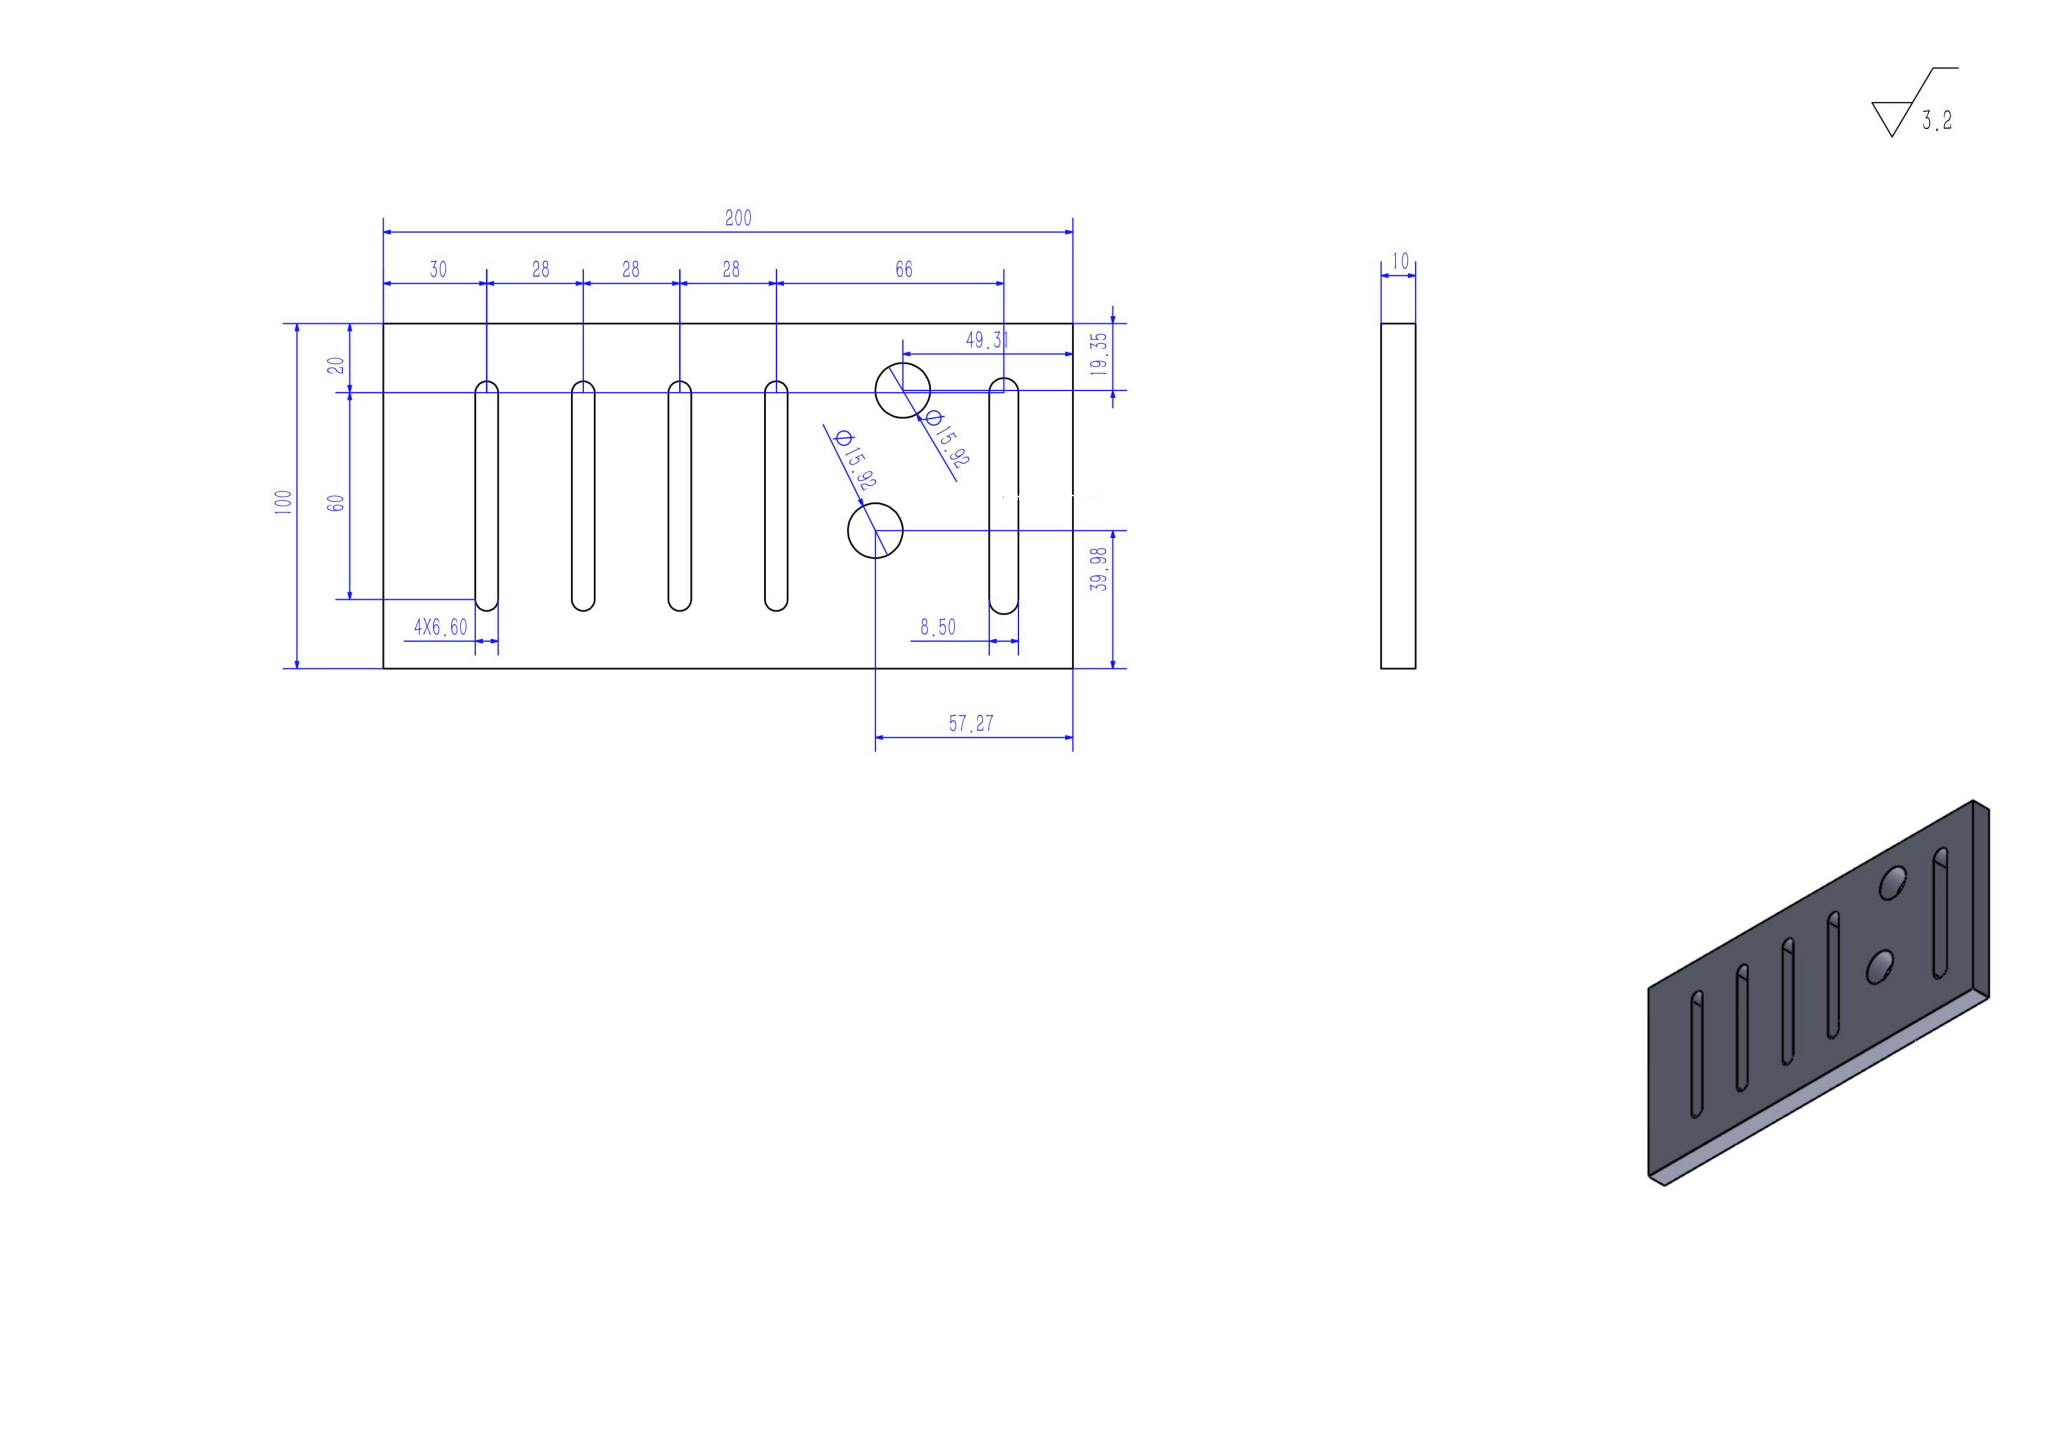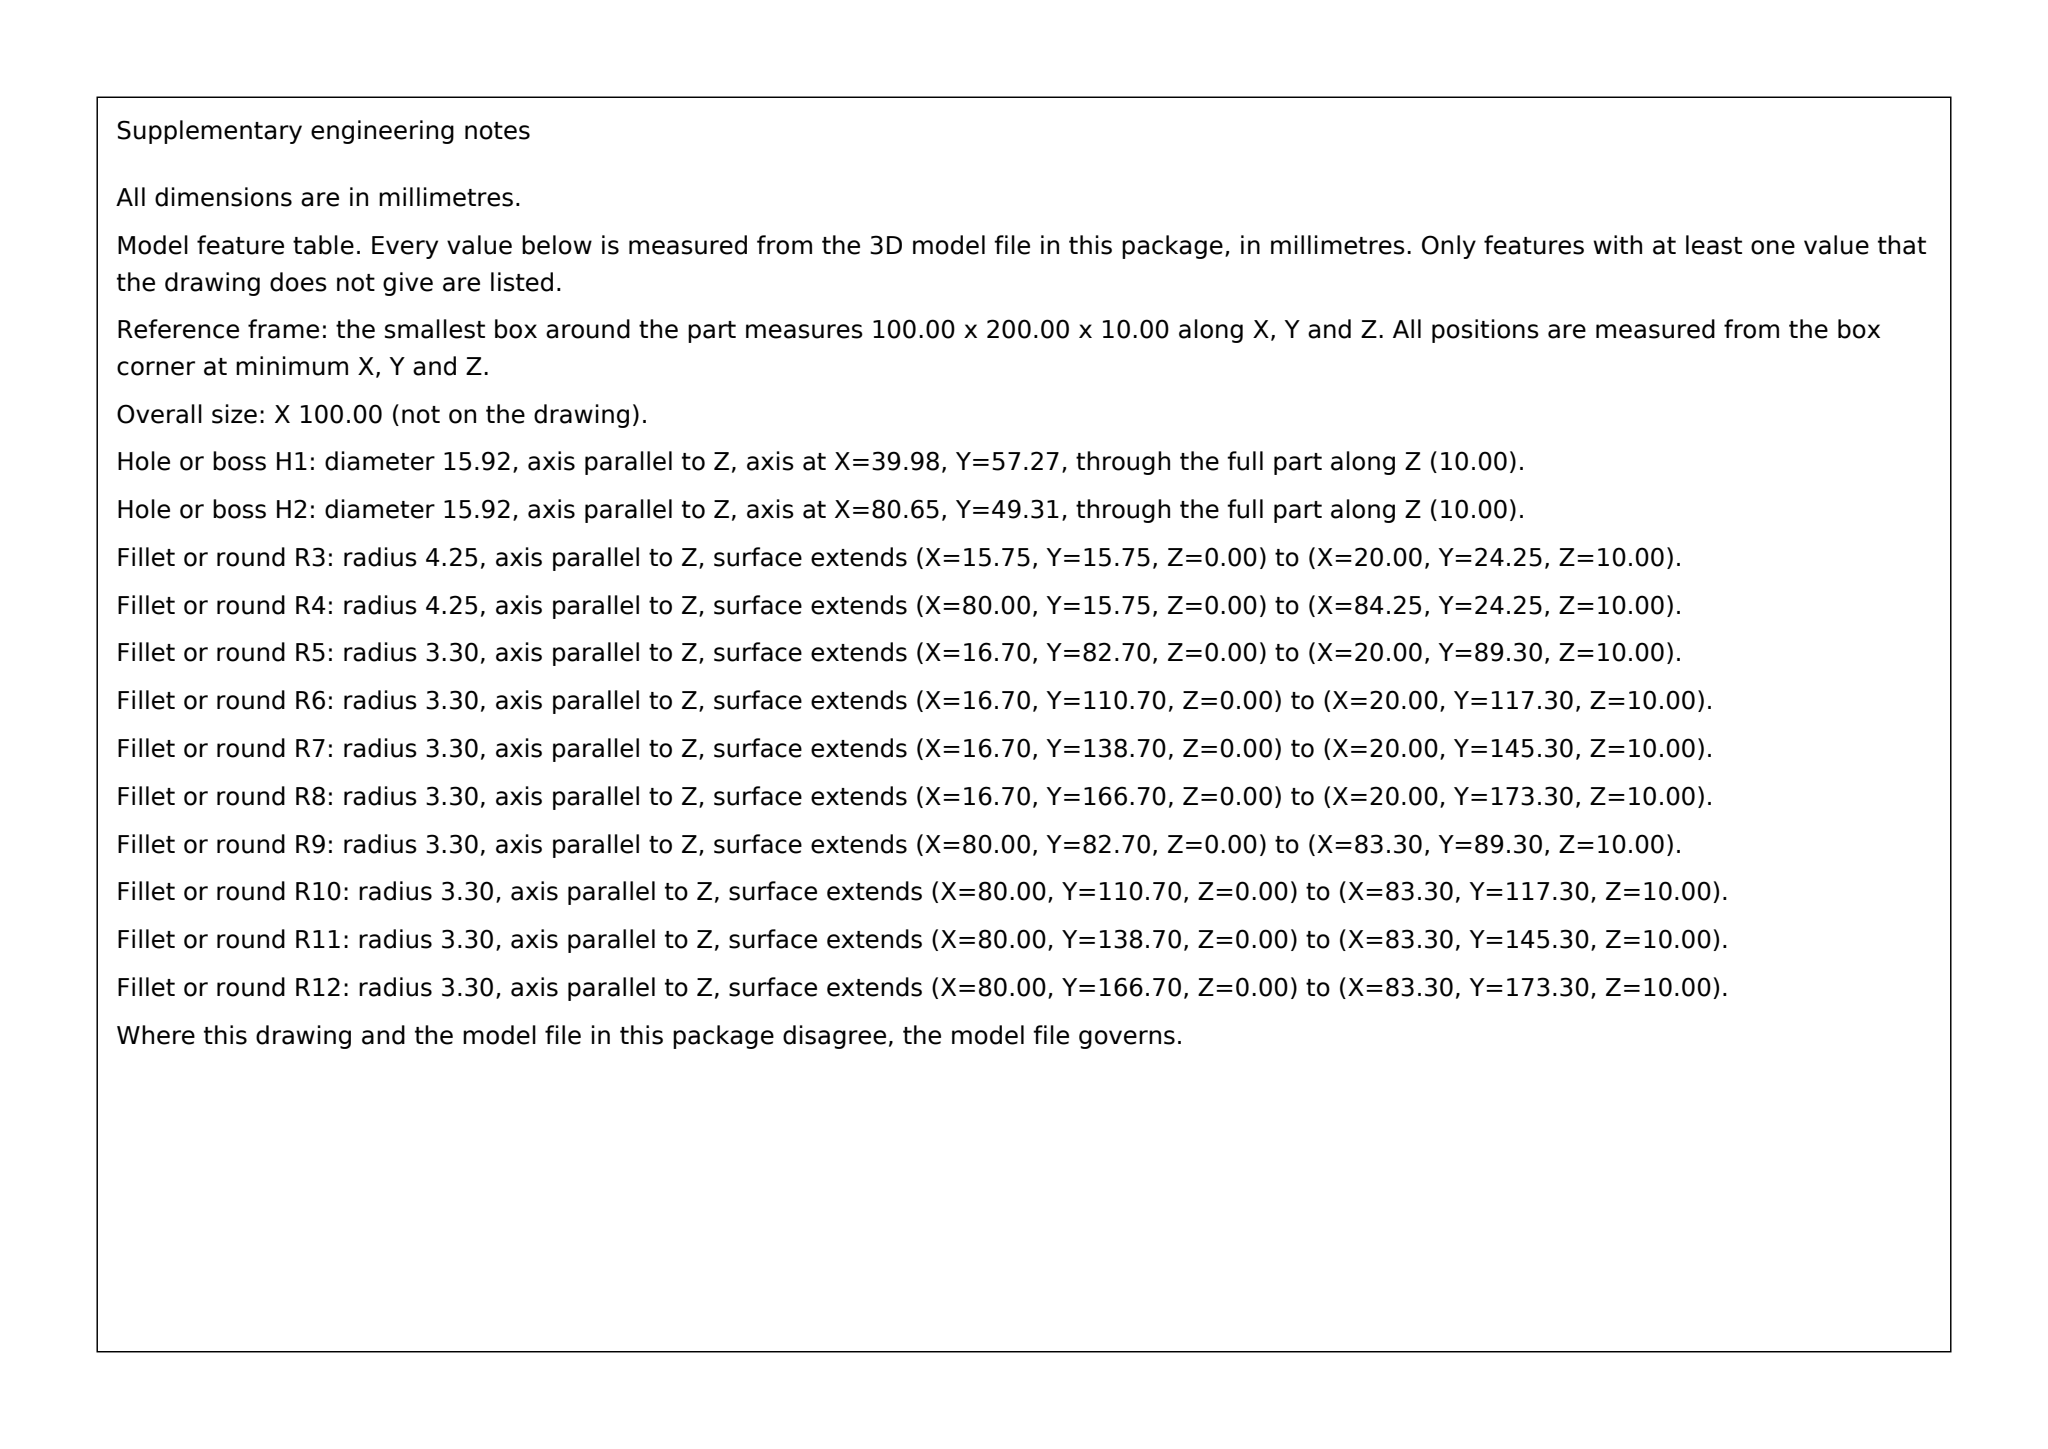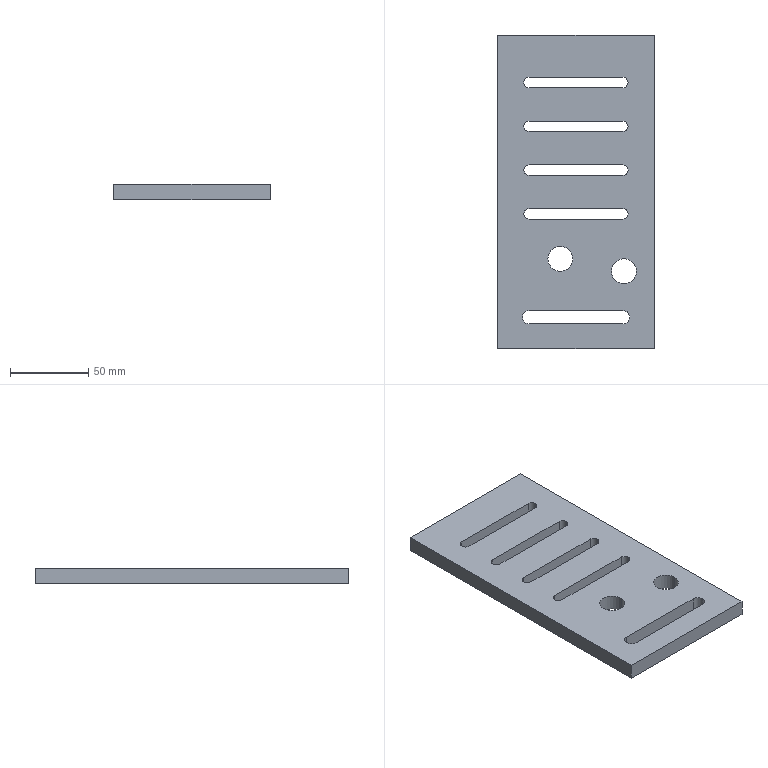Part | SolidWorks | mm | 1 solid | 35 faces | box 100 x 200 x 10 mm | volume 173141 mm3 | cylinder 19 | plane 16 | commonest cylinder face diameters 6.6 x12 15.924 x4 8.5 x3
build123d program:
from build123d import *

# Parameters (mm, degrees)
SKETCH1_W           = 100
SKETCH1_H           = 200
BOSS_EXTRUDE1_DEPTH = 10
CUT_EXTRUDE2_DEPTH  = 10
CUT_EXTRUDE3_DEPTH  = 10
CUT_EXTRUDE4_DEPTH  = 10
SKETCH6_R           = 7.962
CUT_EXTRUDE5_DEPTH  = 80


with BuildPart() as part:
    # Sketch1 → Boss-Extrude1 (new body)
    with BuildSketch(Plane.XY):
        with Locations((500, 81.3)):
            Rectangle(SKETCH1_W, SKETCH1_H)
    extrude(amount=BOSS_EXTRUDE1_DEPTH)

    # Sketch3 → Cut-Extrude2 (cut)
    with BuildSketch(Plane.XY.offset(10)):
        with BuildLine():
            Line((530, 92), (470, 92))
            ThreePointArc((470, 92), (466.7, 95.3), (470, 98.6))
            Line((470, 98.6), (530, 98.6))
            ThreePointArc((530, 98.6), (533.3, 95.3), (530, 92))
        make_face()
        with BuildLine():
            Line((530, 120), (470, 120))
            ThreePointArc((470, 120), (466.7, 123.3), (470, 126.6))
            Line((470, 126.6), (530, 126.6))
            ThreePointArc((530, 126.6), (533.3, 123.3), (530, 120))
        make_face()
        with BuildLine():
            Line((530, 148), (470, 148))
            ThreePointArc((470, 148), (466.7, 151.3), (470, 154.6))
            Line((470, 154.6), (530, 154.6))
            ThreePointArc((530, 154.6), (533.3, 151.3), (530, 148))
        make_face()
    extrude(amount=-CUT_EXTRUDE2_DEPTH, mode=Mode.SUBTRACT)

    # Sketch4 → Cut-Extrude3 (cut)
    with BuildSketch(Plane.XY.offset(10)):
        with BuildLine():
            Line((530, -2.95), (470, -2.95))
            ThreePointArc((470, -2.95), (465.75, 1.3), (470, 5.55))
            Line((470, 5.55), (530, 5.55))
            ThreePointArc((530, 5.55), (534.25, 1.3), (530, -2.95))
        make_face()
    extrude(amount=-CUT_EXTRUDE3_DEPTH, mode=Mode.SUBTRACT)

    # Sketch5 → Cut-Extrude4 (cut)
    with BuildSketch(Plane.XY.offset(10)):
        with BuildLine():
            Line((530, 64), (470, 64))
            ThreePointArc((470, 64), (466.7, 67.3), (470, 70.6))
            Line((470, 70.6), (530, 70.6))
            ThreePointArc((530, 70.6), (533.3, 67.3), (530, 64))
        make_face()
    extrude(amount=-CUT_EXTRUDE4_DEPTH, mode=Mode.SUBTRACT)

    # Sketch6 → Cut-Extrude5 (cut)
    with BuildSketch(Plane.XY.offset(10)):
        with Locations((489.981, 38.571)):
            Circle(SKETCH6_R)
        with Locations((530.647, 30.609)):
            Circle(SKETCH6_R)
    extrude(amount=-CUT_EXTRUDE5_DEPTH, mode=Mode.SUBTRACT)


solid = part.part